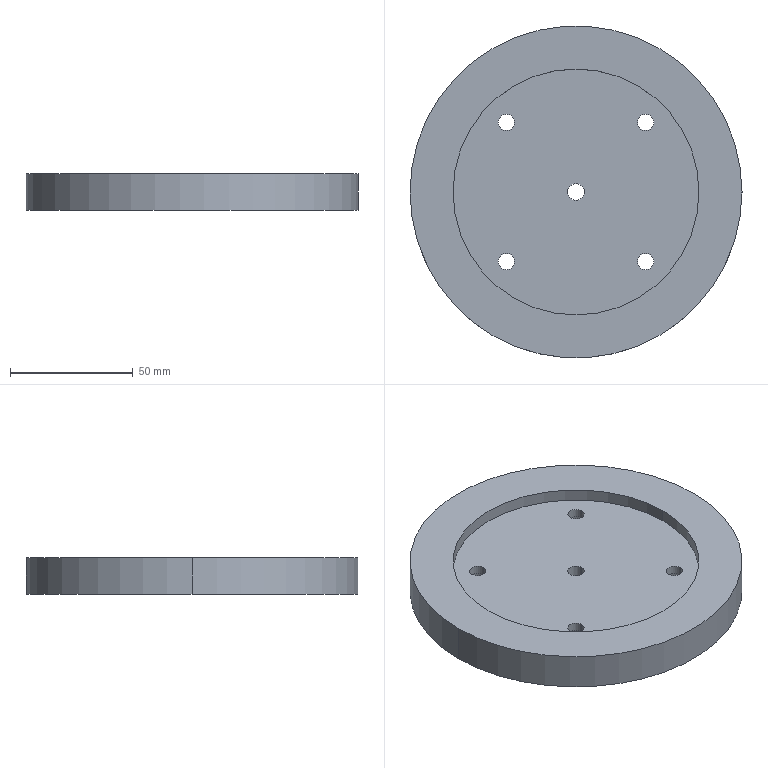Component | SolidWorks | BearingPressingCover-1 | 1 solid | 29 faces | box 135 x 135 x 15 mm | volume 172150 mm3 | cylinder 22 | plane 7 | commonest cylinder face diameters 11 x8 6.6 x8 6.8 x2 100 x2 135 x2 | material 45#
build123d program:
from build123d import *

# Parameters (mm, degrees)
SKETCH1_R                                       = 67.5
BOSS_EXTRUDE1_DEPTH                             = 15
SKETCH2_R                                       = 50
CUT_EXTRUDE1_DEPTH                              = 5
M6_HEX_SOCKET_HEAD_CAP_SCREW_CBORE1_D           = 6.6
M6_HEX_SOCKET_HEAD_CAP_SCREW_CBORE1_CBORE_D     = 11
M6_HEX_SOCKET_HEAD_CAP_SCREW_CBORE1_CBORE_DEPTH = 6.4
M8_TAPPED_HOLE1_D                               = 6.8
M8_TAPPED_HOLE1_DEPTH                           = 19.75
M8_TAPPED_HOLE1_TIP                             = 2.043


with BuildPart() as part:
    # Sketch1 → Boss-Extrude1 (new body)
    with BuildSketch(Plane.XY):
        Circle(SKETCH1_R)
    extrude(amount=BOSS_EXTRUDE1_DEPTH)

    # Sketch2 → Cut-Extrude1 (cut)
    with BuildSketch(Plane.XY.offset(15)):
        Circle(SKETCH2_R)
    extrude(amount=-CUT_EXTRUDE1_DEPTH, mode=Mode.SUBTRACT)

    # M6 Hex Socket Head Cap Screw CBORE1 (through all)
    with Locations(Plane(origin=(28.284, 28.284, 0), x_dir=(-1, 0, 0), z_dir=(0, 0, -1))):
        with Locations((0, 0), (56.569, 0), (56.569, -56.569), (0, -56.569)):
            CounterBoreHole(M6_HEX_SOCKET_HEAD_CAP_SCREW_CBORE1_D / 2, M6_HEX_SOCKET_HEAD_CAP_SCREW_CBORE1_CBORE_D / 2, M6_HEX_SOCKET_HEAD_CAP_SCREW_CBORE1_CBORE_DEPTH)

    # M8 Tapped Hole1
    with Locations(Plane(origin=(0, 0, 0), x_dir=(-1, 0, 0), z_dir=(0, 0, -1))):
        with Locations((0, 0)):
            Hole(M8_TAPPED_HOLE1_D / 2, depth=M8_TAPPED_HOLE1_DEPTH)
            with Locations((0, 0, -(M8_TAPPED_HOLE1_DEPTH + M8_TAPPED_HOLE1_TIP / 2))):  # 118° drill point
                Cone(0, M8_TAPPED_HOLE1_D / 2, M8_TAPPED_HOLE1_TIP, mode=Mode.SUBTRACT)


solid = part.part

# Placed as in the assembly
solid = solid.moved(Location((1.785, -26.917, -1248.21), (0, 0, 0)))
STEP:
#1=COLOUR_RGB('',0.7922,0.8196,0.9333);
#2=FILL_AREA_STYLE_COLOUR('',#1);
#3=FILL_AREA_STYLE('',(#2));
#4=SURFACE_STYLE_FILL_AREA(#3);
#5=SURFACE_SIDE_STYLE('',(#4));
#6=SURFACE_STYLE_USAGE(.BOTH.,#5);
#7=PRESENTATION_STYLE_ASSIGNMENT((#6));
#8=CARTESIAN_POINT('',(0.2041,-1.06,-48.748));
#9=VERTEX_POINT('',#8);
#10=CARTESIAN_POINT('',(-0.06359,-1.06,-48.748));
#11=VERTEX_POINT('',#10);
#12=CARTESIAN_POINT('',(0.07026,-1.06,-48.748));
#13=DIRECTION('',(-0.,0.,1.));
#14=DIRECTION('',(-1.,0.,0.));
#15=AXIS2_PLACEMENT_3D('',#12,#13,#14);
#16=CIRCLE('',#15,0.1339);
#17=EDGE_CURVE('',#9,#11,#16,.T.);
#18=ORIENTED_EDGE('',*,*,#17,.T.);
#19=CARTESIAN_POINT('',(-0.06359,-1.06,-49.142));
#20=VERTEX_POINT('',#19);
#21=CARTESIAN_POINT('',(-0.06359,-1.06,-49.142));
#22=DIRECTION('',(0.,-0.,-1.));
#23=VECTOR('',#22,39.37);
#24=LINE('',#21,#23);
#25=EDGE_CURVE('',#11,#20,#24,.T.);
#26=ORIENTED_EDGE('',*,*,#25,.T.);
#27=CARTESIAN_POINT('',(0.2041,-1.06,-49.142));
#28=VERTEX_POINT('',#27);
#29=CARTESIAN_POINT('',(0.07026,-1.06,-49.142));
#30=DIRECTION('',(0.,-0.,-1.));
#31=DIRECTION('',(1.,0.,0.));
#32=AXIS2_PLACEMENT_3D('',#29,#30,#31);
#33=CIRCLE('',#32,0.1339);
#34=EDGE_CURVE('',#20,#28,#33,.T.);
#35=ORIENTED_EDGE('',*,*,#34,.T.);
#36=CARTESIAN_POINT('',(0.2041,-1.06,-49.142));
#37=DIRECTION('',(0.,-0.,-1.));
#38=VECTOR('',#37,39.37);
#39=LINE('',#36,#38);
#40=EDGE_CURVE('',#9,#28,#39,.T.);
#41=ORIENTED_EDGE('',*,*,#40,.F.);
#42=EDGE_LOOP('',(#18,#26,#35,#41));
#43=FACE_OUTER_BOUND('',#42,.T.);
#44=CARTESIAN_POINT('',(0.07026,-1.06,-49.142));
#45=DIRECTION('',(0.,-0.,-1.));
#46=DIRECTION('',(1.,0.,0.));
#47=AXIS2_PLACEMENT_3D('',#44,#45,#46);
#48=CYLINDRICAL_SURFACE('',#47,0.1339);
#49=ADVANCED_FACE('',(#43),#48,.F.);
#50=CARTESIAN_POINT('',(-1.26,-2.173,-48.89));
#51=VERTEX_POINT('',#50);
#52=CARTESIAN_POINT('',(-0.8268,-2.173,-48.89));
#53=VERTEX_POINT('',#52);
#54=CARTESIAN_POINT('',(-1.043,-2.173,-48.89));
#55=DIRECTION('',(0.,-0.,-1.));
#56=DIRECTION('',(1.,0.,0.));
#57=AXIS2_PLACEMENT_3D('',#54,#55,#56);
#58=CIRCLE('',#57,0.2165);
#59=EDGE_CURVE('',#51,#53,#58,.T.);
#60=ORIENTED_EDGE('',*,*,#59,.F.);
#61=CARTESIAN_POINT('',(-1.26,-2.173,-49.142));
#62=VERTEX_POINT('',#61);
#63=CARTESIAN_POINT('',(-1.26,-2.173,-49.142));
#64=DIRECTION('',(0.,-0.,-1.));
#65=VECTOR('',#64,39.37);
#66=LINE('',#63,#65);
#67=EDGE_CURVE('',#51,#62,#66,.T.);
#68=ORIENTED_EDGE('',*,*,#67,.T.);
#69=CARTESIAN_POINT('',(-0.8268,-2.173,-49.142));
#70=VERTEX_POINT('',#69);
#71=CARTESIAN_POINT('',(-1.043,-2.173,-49.142));
#72=DIRECTION('',(0.,-0.,-1.));
#73=DIRECTION('',(1.,0.,0.));
#74=AXIS2_PLACEMENT_3D('',#71,#72,#73);
#75=CIRCLE('',#74,0.2165);
#76=EDGE_CURVE('',#62,#70,#75,.T.);
#77=ORIENTED_EDGE('',*,*,#76,.T.);
#78=CARTESIAN_POINT('',(-0.8268,-2.173,-49.142));
#79=DIRECTION('',(0.,-0.,-1.));
#80=VECTOR('',#79,39.37);
#81=LINE('',#78,#80);
#82=EDGE_CURVE('',#53,#70,#81,.T.);
#83=ORIENTED_EDGE('',*,*,#82,.F.);
#84=EDGE_LOOP('',(#60,#68,#77,#83));
#85=FACE_OUTER_BOUND('',#84,.T.);
#86=CARTESIAN_POINT('',(-1.043,-2.173,-49.142));
#87=DIRECTION('',(0.,-0.,-1.));
#88=DIRECTION('',(1.,0.,0.));
#89=AXIS2_PLACEMENT_3D('',#86,#87,#88);
#90=CYLINDRICAL_SURFACE('',#89,0.2165);
#91=ADVANCED_FACE('',(#85),#90,.F.);
#92=CARTESIAN_POINT('',(-0.9134,-2.173,-48.748));
#93=VERTEX_POINT('',#92);
#94=CARTESIAN_POINT('',(-1.173,-2.173,-48.748));
#95=VERTEX_POINT('',#94);
#96=CARTESIAN_POINT('',(-1.043,-2.173,-48.748));
#97=DIRECTION('',(-0.,0.,1.));
#98=DIRECTION('',(-1.,0.,0.));
#99=AXIS2_PLACEMENT_3D('',#96,#97,#98);
#100=CIRCLE('',#99,0.1299);
#101=EDGE_CURVE('',#93,#95,#100,.T.);
#102=ORIENTED_EDGE('',*,*,#101,.T.);
#103=CARTESIAN_POINT('',(-1.173,-2.173,-48.89));
#104=VERTEX_POINT('',#103);
#105=CARTESIAN_POINT('',(-1.173,-2.173,-49.142));
#106=DIRECTION('',(0.,-0.,-1.));
#107=VECTOR('',#106,39.37);
#108=LINE('',#105,#107);
#109=EDGE_CURVE('',#95,#104,#108,.T.);
#110=ORIENTED_EDGE('',*,*,#109,.T.);
#111=CARTESIAN_POINT('',(-0.9134,-2.173,-48.89));
#112=VERTEX_POINT('',#111);
#113=CARTESIAN_POINT('',(-1.043,-2.173,-48.89));
#114=DIRECTION('',(0.,-0.,-1.));
#115=DIRECTION('',(1.,0.,0.));
#116=AXIS2_PLACEMENT_3D('',#113,#114,#115);
#117=CIRCLE('',#116,0.1299);
#118=EDGE_CURVE('',#104,#112,#117,.T.);
#119=ORIENTED_EDGE('',*,*,#118,.T.);
#120=CARTESIAN_POINT('',(-0.9134,-2.173,-49.142));
#121=DIRECTION('',(0.,-0.,-1.));
#122=VECTOR('',#121,39.37);
#123=LINE('',#120,#122);
#124=EDGE_CURVE('',#93,#112,#123,.T.);
#125=ORIENTED_EDGE('',*,*,#124,.F.);
#126=EDGE_LOOP('',(#102,#110,#119,#125));
#127=FACE_OUTER_BOUND('',#126,.T.);
#128=CARTESIAN_POINT('',(-1.043,-2.173,-49.142));
#129=DIRECTION('',(0.,-0.,-1.));
#130=DIRECTION('',(1.,0.,0.));
#131=AXIS2_PLACEMENT_3D('',#128,#129,#130);
#132=CYLINDRICAL_SURFACE('',#131,0.1299);
#133=ADVANCED_FACE('',(#127),#132,.F.);
#134=CARTESIAN_POINT('',(0.9673,-2.173,-48.89));
#135=VERTEX_POINT('',#134);
#136=CARTESIAN_POINT('',(1.4,-2.173,-48.89));
#137=VERTEX_POINT('',#136);
#138=CARTESIAN_POINT('',(1.184,-2.173,-48.89));
#139=DIRECTION('',(0.,-0.,-1.));
#140=DIRECTION('',(1.,0.,0.));
#141=AXIS2_PLACEMENT_3D('',#138,#139,#140);
#142=CIRCLE('',#141,0.2165);
#143=EDGE_CURVE('',#135,#137,#142,.T.);
#144=ORIENTED_EDGE('',*,*,#143,.F.);
#145=CARTESIAN_POINT('',(0.9673,-2.173,-49.142));
#146=VERTEX_POINT('',#145);
#147=CARTESIAN_POINT('',(0.9673,-2.173,-49.142));
#148=DIRECTION('',(0.,-0.,-1.));
#149=VECTOR('',#148,39.37);
#150=LINE('',#147,#149);
#151=EDGE_CURVE('',#135,#146,#150,.T.);
#152=ORIENTED_EDGE('',*,*,#151,.T.);
#153=CARTESIAN_POINT('',(1.4,-2.173,-49.142));
#154=VERTEX_POINT('',#153);
#155=CARTESIAN_POINT('',(1.184,-2.173,-49.142));
#156=DIRECTION('',(0.,-0.,-1.));
#157=DIRECTION('',(1.,0.,0.));
#158=AXIS2_PLACEMENT_3D('',#155,#156,#157);
#159=CIRCLE('',#158,0.2165);
#160=EDGE_CURVE('',#146,#154,#159,.T.);
#161=ORIENTED_EDGE('',*,*,#160,.T.);
#162=CARTESIAN_POINT('',(1.4,-2.173,-49.142));
#163=DIRECTION('',(0.,-0.,-1.));
#164=VECTOR('',#163,39.37);
#165=LINE('',#162,#164);
#166=EDGE_CURVE('',#137,#154,#165,.T.);
#167=ORIENTED_EDGE('',*,*,#166,.F.);
#168=EDGE_LOOP('',(#144,#152,#161,#167));
#169=FACE_OUTER_BOUND('',#168,.T.);
#170=CARTESIAN_POINT('',(1.184,-2.173,-49.142));
#171=DIRECTION('',(0.,-0.,-1.));
#172=DIRECTION('',(1.,0.,0.));
#173=AXIS2_PLACEMENT_3D('',#170,#171,#172);
#174=CYLINDRICAL_SURFACE('',#173,0.2165);
#175=ADVANCED_FACE('',(#169),#174,.F.);
#176=CARTESIAN_POINT('',(1.314,-2.173,-48.748));
#177=VERTEX_POINT('',#176);
#178=CARTESIAN_POINT('',(1.054,-2.173,-48.748));
#179=VERTEX_POINT('',#178);
#180=CARTESIAN_POINT('',(1.184,-2.173,-48.748));
#181=DIRECTION('',(-0.,0.,1.));
#182=DIRECTION('',(-1.,0.,0.));
#183=AXIS2_PLACEMENT_3D('',#180,#181,#182);
#184=CIRCLE('',#183,0.1299);
#185=EDGE_CURVE('',#177,#179,#184,.T.);
#186=ORIENTED_EDGE('',*,*,#185,.T.);
#187=CARTESIAN_POINT('',(1.054,-2.173,-48.89));
#188=VERTEX_POINT('',#187);
#189=CARTESIAN_POINT('',(1.054,-2.173,-49.142));
#190=DIRECTION('',(0.,-0.,-1.));
#191=VECTOR('',#190,39.37);
#192=LINE('',#189,#191);
#193=EDGE_CURVE('',#179,#188,#192,.T.);
#194=ORIENTED_EDGE('',*,*,#193,.T.);
#195=CARTESIAN_POINT('',(1.314,-2.173,-48.89));
#196=VERTEX_POINT('',#195);
#197=CARTESIAN_POINT('',(1.184,-2.173,-48.89));
#198=DIRECTION('',(0.,-0.,-1.));
#199=DIRECTION('',(1.,0.,0.));
#200=AXIS2_PLACEMENT_3D('',#197,#198,#199);
#201=CIRCLE('',#200,0.1299);
#202=EDGE_CURVE('',#188,#196,#201,.T.);
#203=ORIENTED_EDGE('',*,*,#202,.T.);
#204=CARTESIAN_POINT('',(1.314,-2.173,-49.142));
#205=DIRECTION('',(0.,-0.,-1.));
#206=VECTOR('',#205,39.37);
#207=LINE('',#204,#206);
#208=EDGE_CURVE('',#177,#196,#207,.T.);
#209=ORIENTED_EDGE('',*,*,#208,.F.);
#210=EDGE_LOOP('',(#186,#194,#203,#209));
#211=FACE_OUTER_BOUND('',#210,.T.);
#212=CARTESIAN_POINT('',(1.184,-2.173,-49.142));
#213=DIRECTION('',(0.,-0.,-1.));
#214=DIRECTION('',(1.,0.,0.));
#215=AXIS2_PLACEMENT_3D('',#212,#213,#214);
#216=CYLINDRICAL_SURFACE('',#215,0.1299);
#217=ADVANCED_FACE('',(#211),#216,.F.);
#218=CARTESIAN_POINT('',(0.9673,0.05383,-48.89));
#219=VERTEX_POINT('',#218);
#220=CARTESIAN_POINT('',(1.4,0.05383,-48.89));
#221=VERTEX_POINT('',#220);
#222=CARTESIAN_POINT('',(1.184,0.05383,-48.89));
#223=DIRECTION('',(0.,-0.,-1.));
#224=DIRECTION('',(1.,-0.,0.));
#225=AXIS2_PLACEMENT_3D('',#222,#223,#224);
#226=CIRCLE('',#225,0.2165);
#227=EDGE_CURVE('',#219,#221,#226,.T.);
#228=ORIENTED_EDGE('',*,*,#227,.F.);
#229=CARTESIAN_POINT('',(0.9673,0.05383,-49.142));
#230=VERTEX_POINT('',#229);
#231=CARTESIAN_POINT('',(0.9673,0.05383,-49.142));
#232=DIRECTION('',(0.,-0.,-1.));
#233=VECTOR('',#232,39.37);
#234=LINE('',#231,#233);
#235=EDGE_CURVE('',#219,#230,#234,.T.);
#236=ORIENTED_EDGE('',*,*,#235,.T.);
#237=CARTESIAN_POINT('',(1.4,0.05383,-49.142));
#238=VERTEX_POINT('',#237);
#239=CARTESIAN_POINT('',(1.184,0.05383,-49.142));
#240=DIRECTION('',(0.,-0.,-1.));
#241=DIRECTION('',(1.,-0.,0.));
#242=AXIS2_PLACEMENT_3D('',#239,#240,#241);
#243=CIRCLE('',#242,0.2165);
#244=EDGE_CURVE('',#230,#238,#243,.T.);
#245=ORIENTED_EDGE('',*,*,#244,.T.);
#246=CARTESIAN_POINT('',(1.4,0.05383,-49.142));
#247=DIRECTION('',(0.,-0.,-1.));
#248=VECTOR('',#247,39.37);
#249=LINE('',#246,#248);
#250=EDGE_CURVE('',#221,#238,#249,.T.);
#251=ORIENTED_EDGE('',*,*,#250,.F.);
#252=EDGE_LOOP('',(#228,#236,#245,#251));
#253=FACE_OUTER_BOUND('',#252,.T.);
#254=CARTESIAN_POINT('',(1.184,0.05383,-49.142));
#255=DIRECTION('',(0.,-0.,-1.));
#256=DIRECTION('',(1.,-0.,0.));
#257=AXIS2_PLACEMENT_3D('',#254,#255,#256);
#258=CYLINDRICAL_SURFACE('',#257,0.2165);
#259=ADVANCED_FACE('',(#253),#258,.F.);
#260=CARTESIAN_POINT('',(1.314,0.05383,-48.748));
#261=VERTEX_POINT('',#260);
#262=CARTESIAN_POINT('',(1.054,0.05383,-48.748));
#263=VERTEX_POINT('',#262);
#264=CARTESIAN_POINT('',(1.184,0.05383,-48.748));
#265=DIRECTION('',(-0.,0.,1.));
#266=DIRECTION('',(-1.,0.,0.));
#267=AXIS2_PLACEMENT_3D('',#264,#265,#266);
#268=CIRCLE('',#267,0.1299);
#269=EDGE_CURVE('',#261,#263,#268,.T.);
#270=ORIENTED_EDGE('',*,*,#269,.T.);
#271=CARTESIAN_POINT('',(1.054,0.05383,-48.89));
#272=VERTEX_POINT('',#271);
#273=CARTESIAN_POINT('',(1.054,0.05383,-49.142));
#274=DIRECTION('',(0.,-0.,-1.));
#275=VECTOR('',#274,39.37);
#276=LINE('',#273,#275);
#277=EDGE_CURVE('',#263,#272,#276,.T.);
#278=ORIENTED_EDGE('',*,*,#277,.T.);
#279=CARTESIAN_POINT('',(1.314,0.05383,-48.89));
#280=VERTEX_POINT('',#279);
#281=CARTESIAN_POINT('',(1.184,0.05383,-48.89));
#282=DIRECTION('',(0.,-0.,-1.));
#283=DIRECTION('',(1.,-0.,0.));
#284=AXIS2_PLACEMENT_3D('',#281,#282,#283);
#285=CIRCLE('',#284,0.1299);
#286=EDGE_CURVE('',#272,#280,#285,.T.);
#287=ORIENTED_EDGE('',*,*,#286,.T.);
#288=CARTESIAN_POINT('',(1.314,0.05383,-49.142));
#289=DIRECTION('',(0.,-0.,-1.));
#290=VECTOR('',#289,39.37);
#291=LINE('',#288,#290);
#292=EDGE_CURVE('',#261,#280,#291,.T.);
#293=ORIENTED_EDGE('',*,*,#292,.F.);
#294=EDGE_LOOP('',(#270,#278,#287,#293));
#295=FACE_OUTER_BOUND('',#294,.T.);
#296=CARTESIAN_POINT('',(1.184,0.05383,-49.142));
#297=DIRECTION('',(0.,-0.,-1.));
#298=DIRECTION('',(1.,-0.,0.));
#299=AXIS2_PLACEMENT_3D('',#296,#297,#298);
#300=CYLINDRICAL_SURFACE('',#299,0.1299);
#301=ADVANCED_FACE('',(#295),#300,.F.);
#302=CARTESIAN_POINT('',(-1.26,0.05383,-48.89));
#303=VERTEX_POINT('',#302);
#304=CARTESIAN_POINT('',(-0.8268,0.05383,-48.89));
#305=VERTEX_POINT('',#304);
#306=CARTESIAN_POINT('',(-1.043,0.05383,-48.89));
#307=DIRECTION('',(0.,-0.,-1.));
#308=DIRECTION('',(1.,-0.,0.));
#309=AXIS2_PLACEMENT_3D('',#306,#307,#308);
#310=CIRCLE('',#309,0.2165);
#311=EDGE_CURVE('',#303,#305,#310,.T.);
#312=ORIENTED_EDGE('',*,*,#311,.F.);
#313=CARTESIAN_POINT('',(-1.26,0.05383,-49.142));
#314=VERTEX_POINT('',#313);
#315=CARTESIAN_POINT('',(-1.26,0.05383,-49.142));
#316=DIRECTION('',(0.,-0.,-1.));
#317=VECTOR('',#316,39.37);
#318=LINE('',#315,#317);
#319=EDGE_CURVE('',#303,#314,#318,.T.);
#320=ORIENTED_EDGE('',*,*,#319,.T.);
#321=CARTESIAN_POINT('',(-0.8268,0.05383,-49.142));
#322=VERTEX_POINT('',#321);
#323=CARTESIAN_POINT('',(-1.043,0.05383,-49.142));
#324=DIRECTION('',(0.,-0.,-1.));
#325=DIRECTION('',(1.,-0.,0.));
#326=AXIS2_PLACEMENT_3D('',#323,#324,#325);
#327=CIRCLE('',#326,0.2165);
#328=EDGE_CURVE('',#314,#322,#327,.T.);
#329=ORIENTED_EDGE('',*,*,#328,.T.);
#330=CARTESIAN_POINT('',(-0.8268,0.05383,-49.142));
#331=DIRECTION('',(0.,-0.,-1.));
#332=VECTOR('',#331,39.37);
#333=LINE('',#330,#332);
#334=EDGE_CURVE('',#305,#322,#333,.T.);
#335=ORIENTED_EDGE('',*,*,#334,.F.);
#336=EDGE_LOOP('',(#312,#320,#329,#335));
#337=FACE_OUTER_BOUND('',#336,.T.);
#338=CARTESIAN_POINT('',(-1.043,0.05383,-49.142));
#339=DIRECTION('',(0.,-0.,-1.));
#340=DIRECTION('',(1.,-0.,0.));
#341=AXIS2_PLACEMENT_3D('',#338,#339,#340);
#342=CYLINDRICAL_SURFACE('',#341,0.2165);
#343=ADVANCED_FACE('',(#337),#342,.F.);
#344=CARTESIAN_POINT('',(-0.9134,0.05383,-48.748));
#345=VERTEX_POINT('',#344);
#346=CARTESIAN_POINT('',(-1.173,0.05383,-48.748));
#347=VERTEX_POINT('',#346);
#348=CARTESIAN_POINT('',(-1.043,0.05383,-48.748));
#349=DIRECTION('',(-0.,0.,1.));
#350=DIRECTION('',(-1.,0.,0.));
#351=AXIS2_PLACEMENT_3D('',#348,#349,#350);
#352=CIRCLE('',#351,0.1299);
#353=EDGE_CURVE('',#345,#347,#352,.T.);
#354=ORIENTED_EDGE('',*,*,#353,.T.);
#355=CARTESIAN_POINT('',(-1.173,0.05383,-48.89));
#356=VERTEX_POINT('',#355);
#357=CARTESIAN_POINT('',(-1.173,0.05383,-49.142));
#358=DIRECTION('',(0.,-0.,-1.));
#359=VECTOR('',#358,39.37);
#360=LINE('',#357,#359);
#361=EDGE_CURVE('',#347,#356,#360,.T.);
#362=ORIENTED_EDGE('',*,*,#361,.T.);
#363=CARTESIAN_POINT('',(-0.9134,0.05383,-48.89));
#364=VERTEX_POINT('',#363);
#365=CARTESIAN_POINT('',(-1.043,0.05383,-48.89));
#366=DIRECTION('',(0.,-0.,-1.));
#367=DIRECTION('',(1.,-0.,0.));
#368=AXIS2_PLACEMENT_3D('',#365,#366,#367);
#369=CIRCLE('',#368,0.1299);
#370=EDGE_CURVE('',#356,#364,#369,.T.);
#371=ORIENTED_EDGE('',*,*,#370,.T.);
#372=CARTESIAN_POINT('',(-0.9134,0.05383,-49.142));
#373=DIRECTION('',(0.,-0.,-1.));
#374=VECTOR('',#373,39.37);
#375=LINE('',#372,#374);
#376=EDGE_CURVE('',#345,#364,#375,.T.);
#377=ORIENTED_EDGE('',*,*,#376,.F.);
#378=EDGE_LOOP('',(#354,#362,#371,#377));
#379=FACE_OUTER_BOUND('',#378,.T.);
#380=CARTESIAN_POINT('',(-1.043,0.05383,-49.142));
#381=DIRECTION('',(0.,-0.,-1.));
#382=DIRECTION('',(1.,-0.,0.));
#383=AXIS2_PLACEMENT_3D('',#380,#381,#382);
#384=CYLINDRICAL_SURFACE('',#383,0.1299);
#385=ADVANCED_FACE('',(#379),#384,.F.);
#386=CARTESIAN_POINT('',(2.039,-1.06,-48.748));
#387=VERTEX_POINT('',#386);
#388=CARTESIAN_POINT('',(-1.898,-1.06,-48.748));
#389=VERTEX_POINT('',#388);
#390=CARTESIAN_POINT('',(0.07026,-1.06,-48.748));
#391=DIRECTION('',(-0.,0.,1.));
#392=DIRECTION('',(-1.,0.,0.));
#393=AXIS2_PLACEMENT_3D('',#390,#391,#392);
#394=CIRCLE('',#393,1.969);
#395=EDGE_CURVE('',#387,#389,#394,.T.);
#396=ORIENTED_EDGE('',*,*,#395,.F.);
#397=CARTESIAN_POINT('',(2.039,-1.06,-48.552));
#398=VERTEX_POINT('',#397);
#399=CARTESIAN_POINT('',(2.039,-1.06,-48.748));
#400=DIRECTION('',(-0.,0.,1.));
#401=VECTOR('',#400,39.37);
#402=LINE('',#399,#401);
#403=EDGE_CURVE('',#387,#398,#402,.T.);
#404=ORIENTED_EDGE('',*,*,#403,.T.);
#405=CARTESIAN_POINT('',(-1.898,-1.06,-48.552));
#406=VERTEX_POINT('',#405);
#407=CARTESIAN_POINT('',(0.07026,-1.06,-48.552));
#408=DIRECTION('',(-0.,0.,1.));
#409=DIRECTION('',(-1.,0.,0.));
#410=AXIS2_PLACEMENT_3D('',#407,#408,#409);
#411=CIRCLE('',#410,1.969);
#412=EDGE_CURVE('',#398,#406,#411,.T.);
#413=ORIENTED_EDGE('',*,*,#412,.T.);
#414=CARTESIAN_POINT('',(-1.898,-1.06,-48.748));
#415=DIRECTION('',(-0.,0.,1.));
#416=VECTOR('',#415,39.37);
#417=LINE('',#414,#416);
#418=EDGE_CURVE('',#389,#406,#417,.T.);
#419=ORIENTED_EDGE('',*,*,#418,.F.);
#420=EDGE_LOOP('',(#396,#404,#413,#419));
#421=FACE_OUTER_BOUND('',#420,.T.);
#422=CARTESIAN_POINT('',(0.07026,-1.06,-48.748));
#423=DIRECTION('',(-0.,0.,1.));
#424=DIRECTION('',(-1.,0.,0.));
#425=AXIS2_PLACEMENT_3D('',#422,#423,#424);
#426=CYLINDRICAL_SURFACE('',#425,1.969);
#427=ADVANCED_FACE('',(#421),#426,.F.);
#428=CARTESIAN_POINT('',(-2.587,-1.06,-48.552));
#429=VERTEX_POINT('',#428);
#430=CARTESIAN_POINT('',(2.728,-1.06,-48.552));
#431=VERTEX_POINT('',#430);
#432=CARTESIAN_POINT('',(0.07026,-1.06,-48.552));
#433=DIRECTION('',(-0.,0.,1.));
#434=DIRECTION('',(-1.,0.,0.));
#435=AXIS2_PLACEMENT_3D('',#432,#433,#434);
#436=CIRCLE('',#435,2.657);
#437=EDGE_CURVE('',#429,#431,#436,.T.);
#438=ORIENTED_EDGE('',*,*,#437,.F.);
#439=CARTESIAN_POINT('',(-2.587,-1.06,-49.142));
#440=VERTEX_POINT('',#439);
#441=CARTESIAN_POINT('',(-2.587,-1.06,-48.552));
#442=DIRECTION('',(0.,-0.,-1.));
#443=VECTOR('',#442,39.37);
#444=LINE('',#441,#443);
#445=EDGE_CURVE('',#429,#440,#444,.T.);
#446=ORIENTED_EDGE('',*,*,#445,.T.);
#447=CARTESIAN_POINT('',(2.728,-1.06,-49.142));
#448=VERTEX_POINT('',#447);
#449=CARTESIAN_POINT('',(0.07026,-1.06,-49.142));
#450=DIRECTION('',(-0.,0.,1.));
#451=DIRECTION('',(-1.,0.,0.));
#452=AXIS2_PLACEMENT_3D('',#449,#450,#451);
#453=CIRCLE('',#452,2.657);
#454=EDGE_CURVE('',#440,#448,#453,.T.);
#455=ORIENTED_EDGE('',*,*,#454,.T.);
#456=CARTESIAN_POINT('',(2.728,-1.06,-48.552));
#457=DIRECTION('',(0.,-0.,-1.));
#458=VECTOR('',#457,39.37);
#459=LINE('',#456,#458);
#460=EDGE_CURVE('',#431,#448,#459,.T.);
#461=ORIENTED_EDGE('',*,*,#460,.F.);
#462=EDGE_LOOP('',(#438,#446,#455,#461));
#463=FACE_OUTER_BOUND('',#462,.T.);
#464=CARTESIAN_POINT('',(0.07026,-1.06,-48.552));
#465=DIRECTION('',(0.,-0.,-1.));
#466=DIRECTION('',(1.,-0.,0.));
#467=AXIS2_PLACEMENT_3D('',#464,#465,#466);
#468=CYLINDRICAL_SURFACE('',#467,2.657);
#469=ADVANCED_FACE('',(#463),#468,.T.);
#470=ORIENTED_EDGE('',*,*,#445,.F.);
#471=CARTESIAN_POINT('',(0.07026,-1.06,-48.552));
#472=DIRECTION('',(-0.,0.,1.));
#473=DIRECTION('',(-1.,0.,0.));
#474=AXIS2_PLACEMENT_3D('',#471,#472,#473);
#475=CIRCLE('',#474,2.657);
#476=EDGE_CURVE('',#431,#429,#475,.T.);
#477=ORIENTED_EDGE('',*,*,#476,.F.);
#478=ORIENTED_EDGE('',*,*,#460,.T.);
#479=CARTESIAN_POINT('',(0.07026,-1.06,-49.142));
#480=DIRECTION('',(-0.,0.,1.));
#481=DIRECTION('',(-1.,0.,0.));
#482=AXIS2_PLACEMENT_3D('',#479,#480,#481);
#483=CIRCLE('',#482,2.657);
#484=EDGE_CURVE('',#448,#440,#483,.T.);
#485=ORIENTED_EDGE('',*,*,#484,.T.);
#486=EDGE_LOOP('',(#470,#477,#478,#485));
#487=FACE_OUTER_BOUND('',#486,.T.);
#488=CARTESIAN_POINT('',(0.07026,-1.06,-48.552));
#489=DIRECTION('',(0.,-0.,-1.));
#490=DIRECTION('',(1.,-0.,0.));
#491=AXIS2_PLACEMENT_3D('',#488,#489,#490);
#492=CYLINDRICAL_SURFACE('',#491,2.657);
#493=ADVANCED_FACE('',(#487),#492,.T.);
#494=CARTESIAN_POINT('',(0.07026,-1.06,-48.552));
#495=DIRECTION('',(-0.,0.,1.));
#496=DIRECTION('',(-1.,0.,0.));
#497=AXIS2_PLACEMENT_3D('',#494,#495,#496);
#498=CIRCLE('',#497,1.969);
#499=EDGE_CURVE('',#406,#398,#498,.T.);
#500=ORIENTED_EDGE('',*,*,#499,.F.);
#501=ORIENTED_EDGE('',*,*,#412,.F.);
#502=EDGE_LOOP('',(#500,#501));
#503=FACE_BOUND('',#502,.T.);
#504=ORIENTED_EDGE('',*,*,#476,.T.);
#505=ORIENTED_EDGE('',*,*,#437,.T.);
#506=EDGE_LOOP('',(#504,#505));
#507=FACE_OUTER_BOUND('',#506,.T.);
#508=CARTESIAN_POINT('',(0.07026,-1.06,-48.552));
#509=DIRECTION('',(-0.,0.,1.));
#510=DIRECTION('',(-1.,0.,-0.));
#511=AXIS2_PLACEMENT_3D('',#508,#509,#510);
#512=PLANE('',#511);
#513=ADVANCED_FACE('',(#503,#507),#512,.T.);
#514=CARTESIAN_POINT('',(0.07026,-1.06,-49.142));
#515=DIRECTION('',(0.,-0.,-1.));
#516=DIRECTION('',(1.,0.,0.));
#517=AXIS2_PLACEMENT_3D('',#514,#515,#516);
#518=CIRCLE('',#517,0.1339);
#519=EDGE_CURVE('',#28,#20,#518,.T.);
#520=ORIENTED_EDGE('',*,*,#519,.F.);
#521=ORIENTED_EDGE('',*,*,#34,.F.);
#522=EDGE_LOOP('',(#520,#521));
#523=FACE_BOUND('',#522,.T.);
#524=CARTESIAN_POINT('',(-1.043,-2.173,-49.142));
#525=DIRECTION('',(0.,-0.,-1.));
#526=DIRECTION('',(1.,0.,0.));
#527=AXIS2_PLACEMENT_3D('',#524,#525,#526);
#528=CIRCLE('',#527,0.2165);
#529=EDGE_CURVE('',#70,#62,#528,.T.);
#530=ORIENTED_EDGE('',*,*,#529,.F.);
#531=ORIENTED_EDGE('',*,*,#76,.F.);
#532=EDGE_LOOP('',(#530,#531));
#533=FACE_BOUND('',#532,.T.);
#534=CARTESIAN_POINT('',(1.184,-2.173,-49.142));
#535=DIRECTION('',(0.,-0.,-1.));
#536=DIRECTION('',(1.,0.,0.));
#537=AXIS2_PLACEMENT_3D('',#534,#535,#536);
#538=CIRCLE('',#537,0.2165);
#539=EDGE_CURVE('',#154,#146,#538,.T.);
#540=ORIENTED_EDGE('',*,*,#539,.F.);
#541=ORIENTED_EDGE('',*,*,#160,.F.);
#542=EDGE_LOOP('',(#540,#541));
#543=FACE_BOUND('',#542,.T.);
#544=CARTESIAN_POINT('',(1.184,0.05383,-49.142));
#545=DIRECTION('',(0.,-0.,-1.));
#546=DIRECTION('',(1.,-0.,0.));
#547=AXIS2_PLACEMENT_3D('',#544,#545,#546);
#548=CIRCLE('',#547,0.2165);
#549=EDGE_CURVE('',#238,#230,#548,.T.);
#550=ORIENTED_EDGE('',*,*,#549,.F.);
#551=ORIENTED_EDGE('',*,*,#244,.F.);
#552=EDGE_LOOP('',(#550,#551));
#553=FACE_BOUND('',#552,.T.);
#554=CARTESIAN_POINT('',(-1.043,0.05383,-49.142));
#555=DIRECTION('',(0.,-0.,-1.));
#556=DIRECTION('',(1.,-0.,0.));
#557=AXIS2_PLACEMENT_3D('',#554,#555,#556);
#558=CIRCLE('',#557,0.2165);
#559=EDGE_CURVE('',#322,#314,#558,.T.);
#560=ORIENTED_EDGE('',*,*,#559,.F.);
#561=ORIENTED_EDGE('',*,*,#328,.F.);
#562=EDGE_LOOP('',(#560,#561));
#563=FACE_BOUND('',#562,.T.);
#564=ORIENTED_EDGE('',*,*,#484,.F.);
#565=ORIENTED_EDGE('',*,*,#454,.F.);
#566=EDGE_LOOP('',(#564,#565));
#567=FACE_OUTER_BOUND('',#566,.T.);
#568=CARTESIAN_POINT('',(0.07026,-1.06,-49.142));
#569=DIRECTION('',(-0.,0.,1.));
#570=DIRECTION('',(-1.,0.,-0.));
#571=AXIS2_PLACEMENT_3D('',#568,#569,#570);
#572=PLANE('',#571);
#573=ADVANCED_FACE('',(#523,#533,#543,#553,#563,#567),#572,.F.);
#574=ORIENTED_EDGE('',*,*,#403,.F.);
#575=CARTESIAN_POINT('',(0.07026,-1.06,-48.748));
#576=DIRECTION('',(-0.,0.,1.));
#577=DIRECTION('',(-1.,0.,0.));
#578=AXIS2_PLACEMENT_3D('',#575,#576,#577);
#579=CIRCLE('',#578,1.969);
#580=EDGE_CURVE('',#389,#387,#579,.T.);
#581=ORIENTED_EDGE('',*,*,#580,.F.);
#582=ORIENTED_EDGE('',*,*,#418,.T.);
#583=ORIENTED_EDGE('',*,*,#499,.T.);
#584=EDGE_LOOP('',(#574,#581,#582,#583));
#585=FACE_OUTER_BOUND('',#584,.T.);
#586=CARTESIAN_POINT('',(0.07026,-1.06,-48.748));
#587=DIRECTION('',(-0.,0.,1.));
#588=DIRECTION('',(-1.,0.,0.));
#589=AXIS2_PLACEMENT_3D('',#586,#587,#588);
#590=CYLINDRICAL_SURFACE('',#589,1.969);
#591=ADVANCED_FACE('',(#585),#590,.F.);
#592=ORIENTED_EDGE('',*,*,#17,.F.);
#593=CARTESIAN_POINT('',(0.07026,-1.06,-48.748));
#594=DIRECTION('',(-0.,0.,1.));
#595=DIRECTION('',(-1.,0.,0.));
#596=AXIS2_PLACEMENT_3D('',#593,#594,#595);
#597=CIRCLE('',#596,0.1339);
#598=EDGE_CURVE('',#11,#9,#597,.T.);
#599=ORIENTED_EDGE('',*,*,#598,.F.);
#600=EDGE_LOOP('',(#592,#599));
#601=FACE_BOUND('',#600,.T.);
#602=ORIENTED_EDGE('',*,*,#101,.F.);
#603=CARTESIAN_POINT('',(-1.043,-2.173,-48.748));
#604=DIRECTION('',(-0.,0.,1.));
#605=DIRECTION('',(-1.,0.,0.));
#606=AXIS2_PLACEMENT_3D('',#603,#604,#605);
#607=CIRCLE('',#606,0.1299);
#608=EDGE_CURVE('',#95,#93,#607,.T.);
#609=ORIENTED_EDGE('',*,*,#608,.F.);
#610=EDGE_LOOP('',(#602,#609));
#611=FACE_BOUND('',#610,.T.);
#612=ORIENTED_EDGE('',*,*,#185,.F.);
#613=CARTESIAN_POINT('',(1.184,-2.173,-48.748));
#614=DIRECTION('',(-0.,0.,1.));
#615=DIRECTION('',(-1.,0.,0.));
#616=AXIS2_PLACEMENT_3D('',#613,#614,#615);
#617=CIRCLE('',#616,0.1299);
#618=EDGE_CURVE('',#179,#177,#617,.T.);
#619=ORIENTED_EDGE('',*,*,#618,.F.);
#620=EDGE_LOOP('',(#612,#619));
#621=FACE_BOUND('',#620,.T.);
#622=ORIENTED_EDGE('',*,*,#269,.F.);
#623=CARTESIAN_POINT('',(1.184,0.05383,-48.748));
#624=DIRECTION('',(-0.,0.,1.));
#625=DIRECTION('',(-1.,0.,0.));
#626=AXIS2_PLACEMENT_3D('',#623,#624,#625);
#627=CIRCLE('',#626,0.1299);
#628=EDGE_CURVE('',#263,#261,#627,.T.);
#629=ORIENTED_EDGE('',*,*,#628,.F.);
#630=EDGE_LOOP('',(#622,#629));
#631=FACE_BOUND('',#630,.T.);
#632=ORIENTED_EDGE('',*,*,#353,.F.);
#633=CARTESIAN_POINT('',(-1.043,0.05383,-48.748));
#634=DIRECTION('',(-0.,0.,1.));
#635=DIRECTION('',(-1.,0.,0.));
#636=AXIS2_PLACEMENT_3D('',#633,#634,#635);
#637=CIRCLE('',#636,0.1299);
#638=EDGE_CURVE('',#347,#345,#637,.T.);
#639=ORIENTED_EDGE('',*,*,#638,.F.);
#640=EDGE_LOOP('',(#632,#639));
#641=FACE_BOUND('',#640,.T.);
#642=ORIENTED_EDGE('',*,*,#580,.T.);
#643=ORIENTED_EDGE('',*,*,#395,.T.);
#644=EDGE_LOOP('',(#642,#643));
#645=FACE_OUTER_BOUND('',#644,.T.);
#646=CARTESIAN_POINT('',(0.07026,-1.06,-48.748));
#647=DIRECTION('',(-0.,0.,1.));
#648=DIRECTION('',(-1.,0.,-0.));
#649=AXIS2_PLACEMENT_3D('',#646,#647,#648);
#650=PLANE('',#649);
#651=ADVANCED_FACE('',(#601,#611,#621,#631,#641,#645),#650,.T.);
#652=ORIENTED_EDGE('',*,*,#361,.F.);
#653=ORIENTED_EDGE('',*,*,#638,.T.);
#654=ORIENTED_EDGE('',*,*,#376,.T.);
#655=CARTESIAN_POINT('',(-1.043,0.05383,-48.89));
#656=DIRECTION('',(0.,-0.,-1.));
#657=DIRECTION('',(1.,-0.,0.));
#658=AXIS2_PLACEMENT_3D('',#655,#656,#657);
#659=CIRCLE('',#658,0.1299);
#660=EDGE_CURVE('',#364,#356,#659,.T.);
#661=ORIENTED_EDGE('',*,*,#660,.T.);
#662=EDGE_LOOP('',(#652,#653,#654,#661));
#663=FACE_OUTER_BOUND('',#662,.T.);
#664=CARTESIAN_POINT('',(-1.043,0.05383,-49.142));
#665=DIRECTION('',(0.,-0.,-1.));
#666=DIRECTION('',(1.,-0.,0.));
#667=AXIS2_PLACEMENT_3D('',#664,#665,#666);
#668=CYLINDRICAL_SURFACE('',#667,0.1299);
#669=ADVANCED_FACE('',(#663),#668,.F.);
#670=ORIENTED_EDGE('',*,*,#660,.F.);
#671=ORIENTED_EDGE('',*,*,#370,.F.);
#672=EDGE_LOOP('',(#670,#671));
#673=FACE_BOUND('',#672,.T.);
#674=CARTESIAN_POINT('',(-1.043,0.05383,-48.89));
#675=DIRECTION('',(0.,-0.,-1.));
#676=DIRECTION('',(1.,-0.,0.));
#677=AXIS2_PLACEMENT_3D('',#674,#675,#676);
#678=CIRCLE('',#677,0.2165);
#679=EDGE_CURVE('',#305,#303,#678,.T.);
#680=ORIENTED_EDGE('',*,*,#679,.T.);
#681=ORIENTED_EDGE('',*,*,#311,.T.);
#682=EDGE_LOOP('',(#680,#681));
#683=FACE_OUTER_BOUND('',#682,.T.);
#684=CARTESIAN_POINT('',(-1.173,0.05383,-48.89));
#685=DIRECTION('',(-0.,0.,1.));
#686=DIRECTION('',(-1.,0.,-0.));
#687=AXIS2_PLACEMENT_3D('',#684,#685,#686);
#688=PLANE('',#687);
#689=ADVANCED_FACE('',(#673,#683),#688,.F.);
#690=ORIENTED_EDGE('',*,*,#319,.F.);
#691=ORIENTED_EDGE('',*,*,#679,.F.);
#692=ORIENTED_EDGE('',*,*,#334,.T.);
#693=ORIENTED_EDGE('',*,*,#559,.T.);
#694=EDGE_LOOP('',(#690,#691,#692,#693));
#695=FACE_OUTER_BOUND('',#694,.T.);
#696=CARTESIAN_POINT('',(-1.043,0.05383,-49.142));
#697=DIRECTION('',(0.,-0.,-1.));
#698=DIRECTION('',(1.,-0.,0.));
#699=AXIS2_PLACEMENT_3D('',#696,#697,#698);
#700=CYLINDRICAL_SURFACE('',#699,0.2165);
#701=ADVANCED_FACE('',(#695),#700,.F.);
#702=ORIENTED_EDGE('',*,*,#277,.F.);
#703=ORIENTED_EDGE('',*,*,#628,.T.);
#704=ORIENTED_EDGE('',*,*,#292,.T.);
#705=CARTESIAN_POINT('',(1.184,0.05383,-48.89));
#706=DIRECTION('',(0.,-0.,-1.));
#707=DIRECTION('',(1.,-0.,0.));
#708=AXIS2_PLACEMENT_3D('',#705,#706,#707);
#709=CIRCLE('',#708,0.1299);
#710=EDGE_CURVE('',#280,#272,#709,.T.);
#711=ORIENTED_EDGE('',*,*,#710,.T.);
#712=EDGE_LOOP('',(#702,#703,#704,#711));
#713=FACE_OUTER_BOUND('',#712,.T.);
#714=CARTESIAN_POINT('',(1.184,0.05383,-49.142));
#715=DIRECTION('',(0.,-0.,-1.));
#716=DIRECTION('',(1.,-0.,0.));
#717=AXIS2_PLACEMENT_3D('',#714,#715,#716);
#718=CYLINDRICAL_SURFACE('',#717,0.1299);
#719=ADVANCED_FACE('',(#713),#718,.F.);
#720=ORIENTED_EDGE('',*,*,#710,.F.);
#721=ORIENTED_EDGE('',*,*,#286,.F.);
#722=EDGE_LOOP('',(#720,#721));
#723=FACE_BOUND('',#722,.T.);
#724=CARTESIAN_POINT('',(1.184,0.05383,-48.89));
#725=DIRECTION('',(0.,-0.,-1.));
#726=DIRECTION('',(1.,-0.,0.));
#727=AXIS2_PLACEMENT_3D('',#724,#725,#726);
#728=CIRCLE('',#727,0.2165);
#729=EDGE_CURVE('',#221,#219,#728,.T.);
#730=ORIENTED_EDGE('',*,*,#729,.T.);
#731=ORIENTED_EDGE('',*,*,#227,.T.);
#732=EDGE_LOOP('',(#730,#731));
#733=FACE_OUTER_BOUND('',#732,.T.);
#734=CARTESIAN_POINT('',(1.054,0.05383,-48.89));
#735=DIRECTION('',(-0.,0.,1.));
#736=DIRECTION('',(-1.,0.,-0.));
#737=AXIS2_PLACEMENT_3D('',#734,#735,#736);
#738=PLANE('',#737);
#739=ADVANCED_FACE('',(#723,#733),#738,.F.);
#740=ORIENTED_EDGE('',*,*,#235,.F.);
#741=ORIENTED_EDGE('',*,*,#729,.F.);
#742=ORIENTED_EDGE('',*,*,#250,.T.);
#743=ORIENTED_EDGE('',*,*,#549,.T.);
#744=EDGE_LOOP('',(#740,#741,#742,#743));
#745=FACE_OUTER_BOUND('',#744,.T.);
#746=CARTESIAN_POINT('',(1.184,0.05383,-49.142));
#747=DIRECTION('',(0.,-0.,-1.));
#748=DIRECTION('',(1.,-0.,0.));
#749=AXIS2_PLACEMENT_3D('',#746,#747,#748);
#750=CYLINDRICAL_SURFACE('',#749,0.2165);
#751=ADVANCED_FACE('',(#745),#750,.F.);
#752=ORIENTED_EDGE('',*,*,#193,.F.);
#753=ORIENTED_EDGE('',*,*,#618,.T.);
#754=ORIENTED_EDGE('',*,*,#208,.T.);
#755=CARTESIAN_POINT('',(1.184,-2.173,-48.89));
#756=DIRECTION('',(0.,-0.,-1.));
#757=DIRECTION('',(1.,0.,0.));
#758=AXIS2_PLACEMENT_3D('',#755,#756,#757);
#759=CIRCLE('',#758,0.1299);
#760=EDGE_CURVE('',#196,#188,#759,.T.);
#761=ORIENTED_EDGE('',*,*,#760,.T.);
#762=EDGE_LOOP('',(#752,#753,#754,#761));
#763=FACE_OUTER_BOUND('',#762,.T.);
#764=CARTESIAN_POINT('',(1.184,-2.173,-49.142));
#765=DIRECTION('',(0.,-0.,-1.));
#766=DIRECTION('',(1.,0.,0.));
#767=AXIS2_PLACEMENT_3D('',#764,#765,#766);
#768=CYLINDRICAL_SURFACE('',#767,0.1299);
#769=ADVANCED_FACE('',(#763),#768,.F.);
#770=ORIENTED_EDGE('',*,*,#760,.F.);
#771=ORIENTED_EDGE('',*,*,#202,.F.);
#772=EDGE_LOOP('',(#770,#771));
#773=FACE_BOUND('',#772,.T.);
#774=CARTESIAN_POINT('',(1.184,-2.173,-48.89));
#775=DIRECTION('',(0.,-0.,-1.));
#776=DIRECTION('',(1.,0.,0.));
#777=AXIS2_PLACEMENT_3D('',#774,#775,#776);
#778=CIRCLE('',#777,0.2165);
#779=EDGE_CURVE('',#137,#135,#778,.T.);
#780=ORIENTED_EDGE('',*,*,#779,.T.);
#781=ORIENTED_EDGE('',*,*,#143,.T.);
#782=EDGE_LOOP('',(#780,#781));
#783=FACE_OUTER_BOUND('',#782,.T.);
#784=CARTESIAN_POINT('',(1.054,-2.173,-48.89));
#785=DIRECTION('',(-0.,0.,1.));
#786=DIRECTION('',(-1.,0.,-0.));
#787=AXIS2_PLACEMENT_3D('',#784,#785,#786);
#788=PLANE('',#787);
#789=ADVANCED_FACE('',(#773,#783),#788,.F.);
#790=ORIENTED_EDGE('',*,*,#151,.F.);
#791=ORIENTED_EDGE('',*,*,#779,.F.);
#792=ORIENTED_EDGE('',*,*,#166,.T.);
#793=ORIENTED_EDGE('',*,*,#539,.T.);
#794=EDGE_LOOP('',(#790,#791,#792,#793));
#795=FACE_OUTER_BOUND('',#794,.T.);
#796=CARTESIAN_POINT('',(1.184,-2.173,-49.142));
#797=DIRECTION('',(0.,-0.,-1.));
#798=DIRECTION('',(1.,0.,0.));
#799=AXIS2_PLACEMENT_3D('',#796,#797,#798);
#800=CYLINDRICAL_SURFACE('',#799,0.2165);
#801=ADVANCED_FACE('',(#795),#800,.F.);
#802=ORIENTED_EDGE('',*,*,#109,.F.);
#803=ORIENTED_EDGE('',*,*,#608,.T.);
#804=ORIENTED_EDGE('',*,*,#124,.T.);
#805=CARTESIAN_POINT('',(-1.043,-2.173,-48.89));
#806=DIRECTION('',(0.,-0.,-1.));
#807=DIRECTION('',(1.,0.,0.));
#808=AXIS2_PLACEMENT_3D('',#805,#806,#807);
#809=CIRCLE('',#808,0.1299);
#810=EDGE_CURVE('',#112,#104,#809,.T.);
#811=ORIENTED_EDGE('',*,*,#810,.T.);
#812=EDGE_LOOP('',(#802,#803,#804,#811));
#813=FACE_OUTER_BOUND('',#812,.T.);
#814=CARTESIAN_POINT('',(-1.043,-2.173,-49.142));
#815=DIRECTION('',(0.,-0.,-1.));
#816=DIRECTION('',(1.,0.,0.));
#817=AXIS2_PLACEMENT_3D('',#814,#815,#816);
#818=CYLINDRICAL_SURFACE('',#817,0.1299);
#819=ADVANCED_FACE('',(#813),#818,.F.);
#820=ORIENTED_EDGE('',*,*,#810,.F.);
#821=ORIENTED_EDGE('',*,*,#118,.F.);
#822=EDGE_LOOP('',(#820,#821));
#823=FACE_BOUND('',#822,.T.);
#824=CARTESIAN_POINT('',(-1.043,-2.173,-48.89));
#825=DIRECTION('',(0.,-0.,-1.));
#826=DIRECTION('',(1.,0.,0.));
#827=AXIS2_PLACEMENT_3D('',#824,#825,#826);
#828=CIRCLE('',#827,0.2165);
#829=EDGE_CURVE('',#53,#51,#828,.T.);
#830=ORIENTED_EDGE('',*,*,#829,.T.);
#831=ORIENTED_EDGE('',*,*,#59,.T.);
#832=EDGE_LOOP('',(#830,#831));
#833=FACE_OUTER_BOUND('',#832,.T.);
#834=CARTESIAN_POINT('',(-1.173,-2.173,-48.89));
#835=DIRECTION('',(-0.,0.,1.));
#836=DIRECTION('',(-1.,0.,-0.));
#837=AXIS2_PLACEMENT_3D('',#834,#835,#836);
#838=PLANE('',#837);
#839=ADVANCED_FACE('',(#823,#833),#838,.F.);
#840=ORIENTED_EDGE('',*,*,#67,.F.);
#841=ORIENTED_EDGE('',*,*,#829,.F.);
#842=ORIENTED_EDGE('',*,*,#82,.T.);
#843=ORIENTED_EDGE('',*,*,#529,.T.);
#844=EDGE_LOOP('',(#840,#841,#842,#843));
#845=FACE_OUTER_BOUND('',#844,.T.);
#846=CARTESIAN_POINT('',(-1.043,-2.173,-49.142));
#847=DIRECTION('',(0.,-0.,-1.));
#848=DIRECTION('',(1.,0.,0.));
#849=AXIS2_PLACEMENT_3D('',#846,#847,#848);
#850=CYLINDRICAL_SURFACE('',#849,0.2165);
#851=ADVANCED_FACE('',(#845),#850,.F.);
#852=ORIENTED_EDGE('',*,*,#25,.F.);
#853=ORIENTED_EDGE('',*,*,#598,.T.);
#854=ORIENTED_EDGE('',*,*,#40,.T.);
#855=ORIENTED_EDGE('',*,*,#519,.T.);
#856=EDGE_LOOP('',(#852,#853,#854,#855));
#857=FACE_OUTER_BOUND('',#856,.T.);
#858=CARTESIAN_POINT('',(0.07026,-1.06,-49.142));
#859=DIRECTION('',(0.,-0.,-1.));
#860=DIRECTION('',(1.,0.,0.));
#861=AXIS2_PLACEMENT_3D('',#858,#859,#860);
#862=CYLINDRICAL_SURFACE('',#861,0.1339);
#863=ADVANCED_FACE('',(#857),#862,.F.);
#864=CLOSED_SHELL('',(#49,#91,#133,#175,#217,#259,#301,#343,#385,#427,#469,#493,#513,#573,#591,#651,#669,#689,#701,#719,#739,#751,#769,#789,#801,#819,#839,#851,#863));
#865=MANIFOLD_SOLID_BREP('',#864);
#866=STYLED_ITEM('',(#7),#865);
#867=(LENGTH_UNIT()NAMED_UNIT(*)SI_UNIT($,.METRE.));
#868=LENGTH_MEASURE_WITH_UNIT(LENGTH_MEASURE(0.0254),#867);
#869=DIMENSIONAL_EXPONENTS(1.,0.,0.,0.,0.,0.,0.);
#870=(CONVERSION_BASED_UNIT('',#868)LENGTH_UNIT()NAMED_UNIT(#869));
#871=UNCERTAINTY_MEASURE_WITH_UNIT(LENGTH_MEASURE(0.00001),#870,'','');
#872=(NAMED_UNIT(*)PLANE_ANGLE_UNIT()SI_UNIT($,.RADIAN.));
#873=(NAMED_UNIT(*)SI_UNIT($,.STERADIAN.)SOLID_ANGLE_UNIT());
#874=(GEOMETRIC_REPRESENTATION_CONTEXT(3)GLOBAL_UNCERTAINTY_ASSIGNED_CONTEXT((#871))GLOBAL_UNIT_ASSIGNED_CONTEXT((#870,#872,#873))REPRESENTATION_CONTEXT('',''));
#875=MECHANICAL_DESIGN_GEOMETRIC_PRESENTATION_REPRESENTATION('',(#866),#874);
#876=CARTESIAN_POINT('',(0.,0.,0.));
#877=DIRECTION('',(0.,0.,1.));
#878=DIRECTION('',(1.,0.,0.));
#879=AXIS2_PLACEMENT_3D('',#876,#877,#878);
#880=(LENGTH_UNIT()NAMED_UNIT(*)SI_UNIT($,.METRE.));
#881=LENGTH_MEASURE_WITH_UNIT(LENGTH_MEASURE(0.0254),#880);
#882=DIMENSIONAL_EXPONENTS(1.,0.,0.,0.,0.,0.,0.);
#883=(CONVERSION_BASED_UNIT('',#881)LENGTH_UNIT()NAMED_UNIT(#882));
#884=UNCERTAINTY_MEASURE_WITH_UNIT(LENGTH_MEASURE(0.00001),#883,'','');
#885=(NAMED_UNIT(*)PLANE_ANGLE_UNIT()SI_UNIT($,.RADIAN.));
#886=(NAMED_UNIT(*)SI_UNIT($,.STERADIAN.)SOLID_ANGLE_UNIT());
#887=(GEOMETRIC_REPRESENTATION_CONTEXT(3)GLOBAL_UNCERTAINTY_ASSIGNED_CONTEXT((#884))GLOBAL_UNIT_ASSIGNED_CONTEXT((#883,#885,#886))REPRESENTATION_CONTEXT('',''));
#888=ADVANCED_BREP_SHAPE_REPRESENTATION('',(#865,#879),#887);
#889=PRESENTATION_LAYER_ASSIGNMENT('','',(#866));